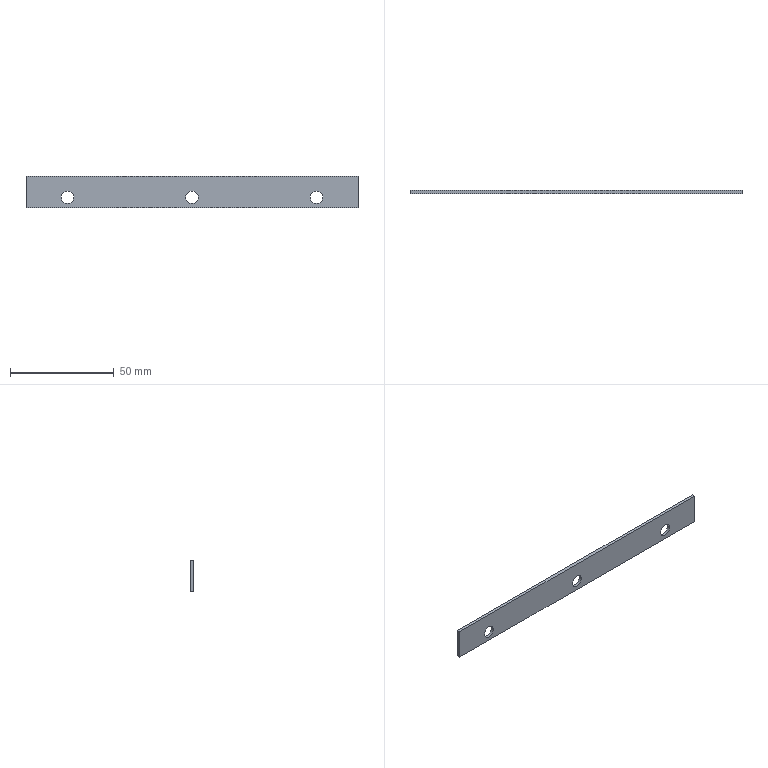Component | SolidWorks | Cover1-7XG1-1 | 1 solid | 12 faces | box 160 x 1.5 x 15 mm | volume 3473 mm3 | cylinder 6 | plane 6 | commonest cylinder face diameters 6 x6
build123d program:
from build123d import *

# Parameters (mm, degrees)
SKETCH1_W           = 160
SKETCH1_H           = 15
BOSS_EXTRUDE1_DEPTH = 1.5
SKETCH2_R           = 3
CUT_EXTRUDE1_DEPTH  = 81.365


with BuildPart() as part:
    # Sketch1 → Boss-Extrude1 (new body)
    with BuildSketch(Plane.XY):
        Rectangle(SKETCH1_W, SKETCH1_H)
    extrude(amount=BOSS_EXTRUDE1_DEPTH)

    # Sketch2 → Cut-Extrude1 (cut, through all)
    with BuildSketch(Plane.XY.offset(1.5)):
        with Locations((-60, -2.5)):
            Circle(SKETCH2_R)
        with Locations((0, -2.5)):
            Circle(SKETCH2_R)
        with Locations((60, -2.5)):
            Circle(SKETCH2_R)
    extrude(amount=-CUT_EXTRUDE1_DEPTH, mode=Mode.SUBTRACT)


solid = part.part

# Placed as in the assembly
solid = solid.moved(Location((0, -153.3, 29), (90, 0, 0)))
STEP:
#1=CARTESIAN_POINT('',(-0.1181,-6.035,1.043));
#2=VERTEX_POINT('',#1);
#3=CARTESIAN_POINT('',(0.1181,-6.035,1.043));
#4=VERTEX_POINT('',#3);
#5=CARTESIAN_POINT('',(-0.,-6.035,1.043));
#6=DIRECTION('',(-0.,-1.,-0.));
#7=DIRECTION('',(1.,0.,0.));
#8=AXIS2_PLACEMENT_3D('',#5,#6,#7);
#9=CIRCLE('',#8,0.1181);
#10=EDGE_CURVE('',#2,#4,#9,.T.);
#11=ORIENTED_EDGE('',*,*,#10,.F.);
#12=CARTESIAN_POINT('',(-0.1181,-6.094,1.043));
#13=VERTEX_POINT('',#12);
#14=CARTESIAN_POINT('',(-0.1181,-6.035,1.043));
#15=DIRECTION('',(-0.,-1.,-0.));
#16=VECTOR('',#15,39.37);
#17=LINE('',#14,#16);
#18=EDGE_CURVE('',#2,#13,#17,.T.);
#19=ORIENTED_EDGE('',*,*,#18,.T.);
#20=CARTESIAN_POINT('',(0.1181,-6.094,1.043));
#21=VERTEX_POINT('',#20);
#22=CARTESIAN_POINT('',(-0.,-6.094,1.043));
#23=DIRECTION('',(-0.,-1.,-0.));
#24=DIRECTION('',(1.,0.,0.));
#25=AXIS2_PLACEMENT_3D('',#22,#23,#24);
#26=CIRCLE('',#25,0.1181);
#27=EDGE_CURVE('',#13,#21,#26,.T.);
#28=ORIENTED_EDGE('',*,*,#27,.T.);
#29=CARTESIAN_POINT('',(0.1181,-6.035,1.043));
#30=DIRECTION('',(-0.,-1.,-0.));
#31=VECTOR('',#30,39.37);
#32=LINE('',#29,#31);
#33=EDGE_CURVE('',#4,#21,#32,.T.);
#34=ORIENTED_EDGE('',*,*,#33,.F.);
#35=EDGE_LOOP('',(#11,#19,#28,#34));
#36=FACE_OUTER_BOUND('',#35,.T.);
#37=CARTESIAN_POINT('',(-0.,-6.035,1.043));
#38=DIRECTION('',(-0.,-1.,-0.));
#39=DIRECTION('',(1.,0.,0.));
#40=AXIS2_PLACEMENT_3D('',#37,#38,#39);
#41=CYLINDRICAL_SURFACE('',#40,0.1181);
#42=ADVANCED_FACE('',(#36),#41,.F.);
#43=CARTESIAN_POINT('',(2.244,-6.035,1.043));
#44=VERTEX_POINT('',#43);
#45=CARTESIAN_POINT('',(2.48,-6.035,1.043));
#46=VERTEX_POINT('',#45);
#47=CARTESIAN_POINT('',(2.362,-6.035,1.043));
#48=DIRECTION('',(-0.,-1.,-0.));
#49=DIRECTION('',(1.,0.,0.));
#50=AXIS2_PLACEMENT_3D('',#47,#48,#49);
#51=CIRCLE('',#50,0.1181);
#52=EDGE_CURVE('',#44,#46,#51,.T.);
#53=ORIENTED_EDGE('',*,*,#52,.F.);
#54=CARTESIAN_POINT('',(2.244,-6.094,1.043));
#55=VERTEX_POINT('',#54);
#56=CARTESIAN_POINT('',(2.244,-6.035,1.043));
#57=DIRECTION('',(-0.,-1.,-0.));
#58=VECTOR('',#57,39.37);
#59=LINE('',#56,#58);
#60=EDGE_CURVE('',#44,#55,#59,.T.);
#61=ORIENTED_EDGE('',*,*,#60,.T.);
#62=CARTESIAN_POINT('',(2.48,-6.094,1.043));
#63=VERTEX_POINT('',#62);
#64=CARTESIAN_POINT('',(2.362,-6.094,1.043));
#65=DIRECTION('',(-0.,-1.,-0.));
#66=DIRECTION('',(1.,0.,0.));
#67=AXIS2_PLACEMENT_3D('',#64,#65,#66);
#68=CIRCLE('',#67,0.1181);
#69=EDGE_CURVE('',#55,#63,#68,.T.);
#70=ORIENTED_EDGE('',*,*,#69,.T.);
#71=CARTESIAN_POINT('',(2.48,-6.035,1.043));
#72=DIRECTION('',(-0.,-1.,-0.));
#73=VECTOR('',#72,39.37);
#74=LINE('',#71,#73);
#75=EDGE_CURVE('',#46,#63,#74,.T.);
#76=ORIENTED_EDGE('',*,*,#75,.F.);
#77=EDGE_LOOP('',(#53,#61,#70,#76));
#78=FACE_OUTER_BOUND('',#77,.T.);
#79=CARTESIAN_POINT('',(2.362,-6.035,1.043));
#80=DIRECTION('',(-0.,-1.,-0.));
#81=DIRECTION('',(1.,0.,0.));
#82=AXIS2_PLACEMENT_3D('',#79,#80,#81);
#83=CYLINDRICAL_SURFACE('',#82,0.1181);
#84=ADVANCED_FACE('',(#78),#83,.F.);
#85=CARTESIAN_POINT('',(-2.48,-6.035,1.043));
#86=VERTEX_POINT('',#85);
#87=CARTESIAN_POINT('',(-2.244,-6.035,1.043));
#88=VERTEX_POINT('',#87);
#89=CARTESIAN_POINT('',(-2.362,-6.035,1.043));
#90=DIRECTION('',(-0.,-1.,-0.));
#91=DIRECTION('',(1.,0.,0.));
#92=AXIS2_PLACEMENT_3D('',#89,#90,#91);
#93=CIRCLE('',#92,0.1181);
#94=EDGE_CURVE('',#86,#88,#93,.T.);
#95=ORIENTED_EDGE('',*,*,#94,.F.);
#96=CARTESIAN_POINT('',(-2.48,-6.094,1.043));
#97=VERTEX_POINT('',#96);
#98=CARTESIAN_POINT('',(-2.48,-6.035,1.043));
#99=DIRECTION('',(-0.,-1.,-0.));
#100=VECTOR('',#99,39.37);
#101=LINE('',#98,#100);
#102=EDGE_CURVE('',#86,#97,#101,.T.);
#103=ORIENTED_EDGE('',*,*,#102,.T.);
#104=CARTESIAN_POINT('',(-2.244,-6.094,1.043));
#105=VERTEX_POINT('',#104);
#106=CARTESIAN_POINT('',(-2.362,-6.094,1.043));
#107=DIRECTION('',(-0.,-1.,-0.));
#108=DIRECTION('',(1.,0.,0.));
#109=AXIS2_PLACEMENT_3D('',#106,#107,#108);
#110=CIRCLE('',#109,0.1181);
#111=EDGE_CURVE('',#97,#105,#110,.T.);
#112=ORIENTED_EDGE('',*,*,#111,.T.);
#113=CARTESIAN_POINT('',(-2.244,-6.035,1.043));
#114=DIRECTION('',(-0.,-1.,-0.));
#115=VECTOR('',#114,39.37);
#116=LINE('',#113,#115);
#117=EDGE_CURVE('',#88,#105,#116,.T.);
#118=ORIENTED_EDGE('',*,*,#117,.F.);
#119=EDGE_LOOP('',(#95,#103,#112,#118));
#120=FACE_OUTER_BOUND('',#119,.T.);
#121=CARTESIAN_POINT('',(-2.362,-6.035,1.043));
#122=DIRECTION('',(-0.,-1.,-0.));
#123=DIRECTION('',(1.,0.,0.));
#124=AXIS2_PLACEMENT_3D('',#121,#122,#123);
#125=CYLINDRICAL_SURFACE('',#124,0.1181);
#126=ADVANCED_FACE('',(#120),#125,.F.);
#127=CARTESIAN_POINT('',(-3.15,-6.035,1.437));
#128=VERTEX_POINT('',#127);
#129=CARTESIAN_POINT('',(-3.15,-6.035,0.8465));
#130=VERTEX_POINT('',#129);
#131=CARTESIAN_POINT('',(-3.15,-6.035,1.437));
#132=DIRECTION('',(0.,0.,-1.));
#133=VECTOR('',#132,39.37);
#134=LINE('',#131,#133);
#135=EDGE_CURVE('',#128,#130,#134,.T.);
#136=ORIENTED_EDGE('',*,*,#135,.T.);
#137=CARTESIAN_POINT('',(-3.15,-6.094,0.8465));
#138=VERTEX_POINT('',#137);
#139=CARTESIAN_POINT('',(-3.15,-6.094,0.8465));
#140=DIRECTION('',(0.,1.,0.));
#141=VECTOR('',#140,39.37);
#142=LINE('',#139,#141);
#143=EDGE_CURVE('',#138,#130,#142,.T.);
#144=ORIENTED_EDGE('',*,*,#143,.F.);
#145=CARTESIAN_POINT('',(-3.15,-6.094,1.437));
#146=VERTEX_POINT('',#145);
#147=CARTESIAN_POINT('',(-3.15,-6.094,1.437));
#148=DIRECTION('',(0.,0.,-1.));
#149=VECTOR('',#148,39.37);
#150=LINE('',#147,#149);
#151=EDGE_CURVE('',#146,#138,#150,.T.);
#152=ORIENTED_EDGE('',*,*,#151,.F.);
#153=CARTESIAN_POINT('',(-3.15,-6.094,1.437));
#154=DIRECTION('',(0.,1.,0.));
#155=VECTOR('',#154,39.37);
#156=LINE('',#153,#155);
#157=EDGE_CURVE('',#146,#128,#156,.T.);
#158=ORIENTED_EDGE('',*,*,#157,.T.);
#159=EDGE_LOOP('',(#136,#144,#152,#158));
#160=FACE_OUTER_BOUND('',#159,.T.);
#161=CARTESIAN_POINT('',(-3.15,-6.094,1.437));
#162=DIRECTION('',(1.,-0.,-0.));
#163=DIRECTION('',(0.,1.,0.));
#164=AXIS2_PLACEMENT_3D('',#161,#162,#163);
#165=PLANE('',#164);
#166=ADVANCED_FACE('',(#160),#165,.F.);
#167=CARTESIAN_POINT('',(3.15,-6.035,0.8465));
#168=VERTEX_POINT('',#167);
#169=CARTESIAN_POINT('',(-3.15,-6.035,0.8465));
#170=DIRECTION('',(1.,-0.,-0.));
#171=VECTOR('',#170,39.37);
#172=LINE('',#169,#171);
#173=EDGE_CURVE('',#130,#168,#172,.T.);
#174=ORIENTED_EDGE('',*,*,#173,.T.);
#175=CARTESIAN_POINT('',(3.15,-6.094,0.8465));
#176=VERTEX_POINT('',#175);
#177=CARTESIAN_POINT('',(3.15,-6.094,0.8465));
#178=DIRECTION('',(0.,1.,0.));
#179=VECTOR('',#178,39.37);
#180=LINE('',#177,#179);
#181=EDGE_CURVE('',#176,#168,#180,.T.);
#182=ORIENTED_EDGE('',*,*,#181,.F.);
#183=CARTESIAN_POINT('',(-3.15,-6.094,0.8465));
#184=DIRECTION('',(1.,-0.,-0.));
#185=VECTOR('',#184,39.37);
#186=LINE('',#183,#185);
#187=EDGE_CURVE('',#138,#176,#186,.T.);
#188=ORIENTED_EDGE('',*,*,#187,.F.);
#189=ORIENTED_EDGE('',*,*,#143,.T.);
#190=EDGE_LOOP('',(#174,#182,#188,#189));
#191=FACE_OUTER_BOUND('',#190,.T.);
#192=CARTESIAN_POINT('',(-3.15,-6.094,0.8465));
#193=DIRECTION('',(-0.,-0.,1.));
#194=DIRECTION('',(-0.,-1.,-0.));
#195=AXIS2_PLACEMENT_3D('',#192,#193,#194);
#196=PLANE('',#195);
#197=ADVANCED_FACE('',(#191),#196,.F.);
#198=CARTESIAN_POINT('',(3.15,-6.035,1.437));
#199=VERTEX_POINT('',#198);
#200=CARTESIAN_POINT('',(3.15,-6.035,1.437));
#201=DIRECTION('',(-0.,-0.,1.));
#202=VECTOR('',#201,39.37);
#203=LINE('',#200,#202);
#204=EDGE_CURVE('',#168,#199,#203,.T.);
#205=ORIENTED_EDGE('',*,*,#204,.T.);
#206=CARTESIAN_POINT('',(3.15,-6.094,1.437));
#207=VERTEX_POINT('',#206);
#208=CARTESIAN_POINT('',(3.15,-6.094,1.437));
#209=DIRECTION('',(0.,1.,0.));
#210=VECTOR('',#209,39.37);
#211=LINE('',#208,#210);
#212=EDGE_CURVE('',#207,#199,#211,.T.);
#213=ORIENTED_EDGE('',*,*,#212,.F.);
#214=CARTESIAN_POINT('',(3.15,-6.094,1.437));
#215=DIRECTION('',(-0.,-0.,1.));
#216=VECTOR('',#215,39.37);
#217=LINE('',#214,#216);
#218=EDGE_CURVE('',#176,#207,#217,.T.);
#219=ORIENTED_EDGE('',*,*,#218,.F.);
#220=ORIENTED_EDGE('',*,*,#181,.T.);
#221=EDGE_LOOP('',(#205,#213,#219,#220));
#222=FACE_OUTER_BOUND('',#221,.T.);
#223=CARTESIAN_POINT('',(3.15,-6.094,1.437));
#224=DIRECTION('',(-1.,0.,0.));
#225=DIRECTION('',(-0.,-1.,-0.));
#226=AXIS2_PLACEMENT_3D('',#223,#224,#225);
#227=PLANE('',#226);
#228=ADVANCED_FACE('',(#222),#227,.F.);
#229=CARTESIAN_POINT('',(-3.15,-6.035,1.437));
#230=DIRECTION('',(-1.,0.,0.));
#231=VECTOR('',#230,39.37);
#232=LINE('',#229,#231);
#233=EDGE_CURVE('',#199,#128,#232,.T.);
#234=ORIENTED_EDGE('',*,*,#233,.T.);
#235=ORIENTED_EDGE('',*,*,#157,.F.);
#236=CARTESIAN_POINT('',(-3.15,-6.094,1.437));
#237=DIRECTION('',(-1.,0.,0.));
#238=VECTOR('',#237,39.37);
#239=LINE('',#236,#238);
#240=EDGE_CURVE('',#207,#146,#239,.T.);
#241=ORIENTED_EDGE('',*,*,#240,.F.);
#242=ORIENTED_EDGE('',*,*,#212,.T.);
#243=EDGE_LOOP('',(#234,#235,#241,#242));
#244=FACE_OUTER_BOUND('',#243,.T.);
#245=CARTESIAN_POINT('',(-3.15,-6.094,1.437));
#246=DIRECTION('',(0.,0.,-1.));
#247=DIRECTION('',(0.,1.,0.));
#248=AXIS2_PLACEMENT_3D('',#245,#246,#247);
#249=PLANE('',#248);
#250=ADVANCED_FACE('',(#244),#249,.F.);
#251=CARTESIAN_POINT('',(-0.,-6.094,1.043));
#252=DIRECTION('',(-0.,-1.,-0.));
#253=DIRECTION('',(1.,0.,0.));
#254=AXIS2_PLACEMENT_3D('',#251,#252,#253);
#255=CIRCLE('',#254,0.1181);
#256=EDGE_CURVE('',#21,#13,#255,.T.);
#257=ORIENTED_EDGE('',*,*,#256,.F.);
#258=ORIENTED_EDGE('',*,*,#27,.F.);
#259=EDGE_LOOP('',(#257,#258));
#260=FACE_BOUND('',#259,.T.);
#261=CARTESIAN_POINT('',(2.362,-6.094,1.043));
#262=DIRECTION('',(-0.,-1.,-0.));
#263=DIRECTION('',(1.,0.,0.));
#264=AXIS2_PLACEMENT_3D('',#261,#262,#263);
#265=CIRCLE('',#264,0.1181);
#266=EDGE_CURVE('',#63,#55,#265,.T.);
#267=ORIENTED_EDGE('',*,*,#266,.F.);
#268=ORIENTED_EDGE('',*,*,#69,.F.);
#269=EDGE_LOOP('',(#267,#268));
#270=FACE_BOUND('',#269,.T.);
#271=CARTESIAN_POINT('',(-2.362,-6.094,1.043));
#272=DIRECTION('',(-0.,-1.,-0.));
#273=DIRECTION('',(1.,0.,0.));
#274=AXIS2_PLACEMENT_3D('',#271,#272,#273);
#275=CIRCLE('',#274,0.1181);
#276=EDGE_CURVE('',#105,#97,#275,.T.);
#277=ORIENTED_EDGE('',*,*,#276,.F.);
#278=ORIENTED_EDGE('',*,*,#111,.F.);
#279=EDGE_LOOP('',(#277,#278));
#280=FACE_BOUND('',#279,.T.);
#281=ORIENTED_EDGE('',*,*,#151,.T.);
#282=ORIENTED_EDGE('',*,*,#187,.T.);
#283=ORIENTED_EDGE('',*,*,#218,.T.);
#284=ORIENTED_EDGE('',*,*,#240,.T.);
#285=EDGE_LOOP('',(#281,#282,#283,#284));
#286=FACE_OUTER_BOUND('',#285,.T.);
#287=CARTESIAN_POINT('',(-0.,-6.094,1.142));
#288=DIRECTION('',(-0.,-1.,-0.));
#289=DIRECTION('',(1.,-0.,-0.));
#290=AXIS2_PLACEMENT_3D('',#287,#288,#289);
#291=PLANE('',#290);
#292=ADVANCED_FACE('',(#260,#270,#280,#286),#291,.T.);
#293=CARTESIAN_POINT('',(-0.,-6.035,1.043));
#294=DIRECTION('',(-0.,-1.,-0.));
#295=DIRECTION('',(1.,0.,0.));
#296=AXIS2_PLACEMENT_3D('',#293,#294,#295);
#297=CIRCLE('',#296,0.1181);
#298=EDGE_CURVE('',#4,#2,#297,.T.);
#299=ORIENTED_EDGE('',*,*,#298,.T.);
#300=ORIENTED_EDGE('',*,*,#10,.T.);
#301=EDGE_LOOP('',(#299,#300));
#302=FACE_BOUND('',#301,.T.);
#303=CARTESIAN_POINT('',(2.362,-6.035,1.043));
#304=DIRECTION('',(-0.,-1.,-0.));
#305=DIRECTION('',(1.,0.,0.));
#306=AXIS2_PLACEMENT_3D('',#303,#304,#305);
#307=CIRCLE('',#306,0.1181);
#308=EDGE_CURVE('',#46,#44,#307,.T.);
#309=ORIENTED_EDGE('',*,*,#308,.T.);
#310=ORIENTED_EDGE('',*,*,#52,.T.);
#311=EDGE_LOOP('',(#309,#310));
#312=FACE_BOUND('',#311,.T.);
#313=CARTESIAN_POINT('',(-2.362,-6.035,1.043));
#314=DIRECTION('',(-0.,-1.,-0.));
#315=DIRECTION('',(1.,0.,0.));
#316=AXIS2_PLACEMENT_3D('',#313,#314,#315);
#317=CIRCLE('',#316,0.1181);
#318=EDGE_CURVE('',#88,#86,#317,.T.);
#319=ORIENTED_EDGE('',*,*,#318,.T.);
#320=ORIENTED_EDGE('',*,*,#94,.T.);
#321=EDGE_LOOP('',(#319,#320));
#322=FACE_BOUND('',#321,.T.);
#323=ORIENTED_EDGE('',*,*,#135,.F.);
#324=ORIENTED_EDGE('',*,*,#233,.F.);
#325=ORIENTED_EDGE('',*,*,#204,.F.);
#326=ORIENTED_EDGE('',*,*,#173,.F.);
#327=EDGE_LOOP('',(#323,#324,#325,#326));
#328=FACE_OUTER_BOUND('',#327,.T.);
#329=CARTESIAN_POINT('',(-0.,-6.035,1.142));
#330=DIRECTION('',(-0.,-1.,-0.));
#331=DIRECTION('',(1.,-0.,-0.));
#332=AXIS2_PLACEMENT_3D('',#329,#330,#331);
#333=PLANE('',#332);
#334=ADVANCED_FACE('',(#302,#312,#322,#328),#333,.F.);
#335=ORIENTED_EDGE('',*,*,#102,.F.);
#336=ORIENTED_EDGE('',*,*,#318,.F.);
#337=ORIENTED_EDGE('',*,*,#117,.T.);
#338=ORIENTED_EDGE('',*,*,#276,.T.);
#339=EDGE_LOOP('',(#335,#336,#337,#338));
#340=FACE_OUTER_BOUND('',#339,.T.);
#341=CARTESIAN_POINT('',(-2.362,-6.035,1.043));
#342=DIRECTION('',(-0.,-1.,-0.));
#343=DIRECTION('',(1.,0.,0.));
#344=AXIS2_PLACEMENT_3D('',#341,#342,#343);
#345=CYLINDRICAL_SURFACE('',#344,0.1181);
#346=ADVANCED_FACE('',(#340),#345,.F.);
#347=ORIENTED_EDGE('',*,*,#60,.F.);
#348=ORIENTED_EDGE('',*,*,#308,.F.);
#349=ORIENTED_EDGE('',*,*,#75,.T.);
#350=ORIENTED_EDGE('',*,*,#266,.T.);
#351=EDGE_LOOP('',(#347,#348,#349,#350));
#352=FACE_OUTER_BOUND('',#351,.T.);
#353=CARTESIAN_POINT('',(2.362,-6.035,1.043));
#354=DIRECTION('',(-0.,-1.,-0.));
#355=DIRECTION('',(1.,0.,0.));
#356=AXIS2_PLACEMENT_3D('',#353,#354,#355);
#357=CYLINDRICAL_SURFACE('',#356,0.1181);
#358=ADVANCED_FACE('',(#352),#357,.F.);
#359=ORIENTED_EDGE('',*,*,#18,.F.);
#360=ORIENTED_EDGE('',*,*,#298,.F.);
#361=ORIENTED_EDGE('',*,*,#33,.T.);
#362=ORIENTED_EDGE('',*,*,#256,.T.);
#363=EDGE_LOOP('',(#359,#360,#361,#362));
#364=FACE_OUTER_BOUND('',#363,.T.);
#365=CARTESIAN_POINT('',(-0.,-6.035,1.043));
#366=DIRECTION('',(-0.,-1.,-0.));
#367=DIRECTION('',(1.,0.,0.));
#368=AXIS2_PLACEMENT_3D('',#365,#366,#367);
#369=CYLINDRICAL_SURFACE('',#368,0.1181);
#370=ADVANCED_FACE('',(#364),#369,.F.);
#371=CLOSED_SHELL('',(#42,#84,#126,#166,#197,#228,#250,#292,#334,#346,#358,#370));
#372=MANIFOLD_SOLID_BREP('',#371);
#373=CARTESIAN_POINT('',(0.,0.,0.));
#374=DIRECTION('',(0.,0.,1.));
#375=DIRECTION('',(1.,0.,0.));
#376=AXIS2_PLACEMENT_3D('',#373,#374,#375);
#377=(LENGTH_UNIT()NAMED_UNIT(*)SI_UNIT($,.METRE.));
#378=LENGTH_MEASURE_WITH_UNIT(LENGTH_MEASURE(0.0254),#377);
#379=DIMENSIONAL_EXPONENTS(1.,0.,0.,0.,0.,0.,0.);
#380=(CONVERSION_BASED_UNIT('',#378)LENGTH_UNIT()NAMED_UNIT(#379));
#381=UNCERTAINTY_MEASURE_WITH_UNIT(LENGTH_MEASURE(0.00001),#380,'','');
#382=(NAMED_UNIT(*)PLANE_ANGLE_UNIT()SI_UNIT($,.RADIAN.));
#383=(NAMED_UNIT(*)SI_UNIT($,.STERADIAN.)SOLID_ANGLE_UNIT());
#384=(GEOMETRIC_REPRESENTATION_CONTEXT(3)GLOBAL_UNCERTAINTY_ASSIGNED_CONTEXT((#381))GLOBAL_UNIT_ASSIGNED_CONTEXT((#380,#382,#383))REPRESENTATION_CONTEXT('',''));
#385=ADVANCED_BREP_SHAPE_REPRESENTATION('',(#372,#376),#384);
#386=COLOUR_RGB('',0.7922,0.8196,0.9333);
#387=FILL_AREA_STYLE_COLOUR('',#386);
#388=FILL_AREA_STYLE('',(#387));
#389=SURFACE_STYLE_FILL_AREA(#388);
#390=SURFACE_SIDE_STYLE('',(#389));
#391=SURFACE_STYLE_USAGE(.BOTH.,#390);
#392=PRESENTATION_STYLE_ASSIGNMENT((#391));
#393=STYLED_ITEM('',(#392),#372);
#394=(LENGTH_UNIT()NAMED_UNIT(*)SI_UNIT($,.METRE.));
#395=LENGTH_MEASURE_WITH_UNIT(LENGTH_MEASURE(0.0254),#394);
#396=DIMENSIONAL_EXPONENTS(1.,0.,0.,0.,0.,0.,0.);
#397=(CONVERSION_BASED_UNIT('',#395)LENGTH_UNIT()NAMED_UNIT(#396));
#398=UNCERTAINTY_MEASURE_WITH_UNIT(LENGTH_MEASURE(0.00001),#397,'','');
#399=(NAMED_UNIT(*)PLANE_ANGLE_UNIT()SI_UNIT($,.RADIAN.));
#400=(NAMED_UNIT(*)SI_UNIT($,.STERADIAN.)SOLID_ANGLE_UNIT());
#401=(GEOMETRIC_REPRESENTATION_CONTEXT(3)GLOBAL_UNCERTAINTY_ASSIGNED_CONTEXT((#398))GLOBAL_UNIT_ASSIGNED_CONTEXT((#397,#399,#400))REPRESENTATION_CONTEXT('',''));
#402=MECHANICAL_DESIGN_GEOMETRIC_PRESENTATION_REPRESENTATION('',(#393),#401);
#403=PRESENTATION_LAYER_ASSIGNMENT('','',(#393));